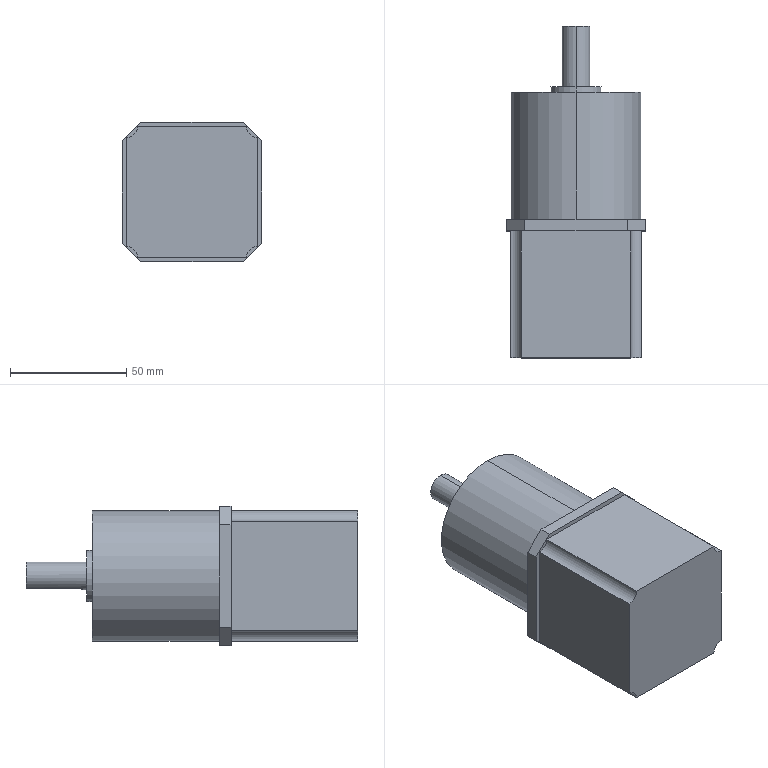Component | SolidWorks | LatestStepperMotor-1 | 1 solid | 49 faces | box 60 x 142.5 x 60 mm | volume 321837 mm3 | plane 21 | cylinder 20 | cone 8 | commonest cylinder face diameters 4.2 x8 9 x4 5 x2 12 x2 21.95 x2 56 x2 | material AISI 1045 Steel, Cold Drawn
build123d program:
from build123d import *

# Parameters (mm, degrees)
BOSS_EXTRUDE1_DEPTH   = 27.25
SKETCH2_W             = 60
SKETCH2_H             = 60
BOSS_EXTRUDE2_DEPTH   = 5
SKETCH3_R             = 28
BOSS_EXTRUDE3_DEPTH   = 54.5
SKETCH4_R             = 10.975
BOSS_EXTRUDE4_DEPTH   = 2.5
SKETCH5_R             = 6
BOSS_EXTRUDE5_DEPTH   = 26
CHAMFER1_SIZE         = 8
M5_TAPPED_HOLE1_D     = 4.2
M5_TAPPED_HOLE1_DEPTH = 13
M5_TAPPED_HOLE1_TIP   = 1.212
CUT_EXTRUDE1_DEPTH    = 3


with BuildPart() as part:
    # Sketch1 → Boss-Extrude1 (new, symmetric)
    with BuildSketch(Plane.XY):
        with BuildLine():
            Line((-23.5, 28), (23.5, 28))
            ThreePointArc((23.5, 28), (24.818, 24.818), (28, 23.5))
            Line((28, 23.5), (28, -23.5))
            ThreePointArc((28, -23.5), (24.818, -24.818), (23.5, -28))
            Line((23.5, -28), (-23.5, -28))
            ThreePointArc((-23.5, -28), (-24.818, -24.818), (-28, -23.5))
            Line((-28, -23.5), (-28, 23.5))
            ThreePointArc((-28, 23.5), (-24.818, 24.818), (-23.5, 28))
        make_face()
    extrude(amount=BOSS_EXTRUDE1_DEPTH, both=True)

    # Sketch2 → Boss-Extrude2 (add)
    with BuildSketch(Plane.XY.offset(27.25)):
        Rectangle(SKETCH2_W, SKETCH2_H)
    extrude(amount=BOSS_EXTRUDE2_DEPTH)

    # Sketch3 → Boss-Extrude3 (add)
    with BuildSketch(Plane.XY.offset(32.25)):
        Circle(SKETCH3_R)
    extrude(amount=BOSS_EXTRUDE3_DEPTH)

    # Sketch4 → Boss-Extrude4 (add)
    with BuildSketch(Plane.XY.offset(86.75)):
        Circle(SKETCH4_R)
    extrude(amount=BOSS_EXTRUDE4_DEPTH)

    # Sketch5 → Boss-Extrude5 (add)
    with BuildSketch(Plane.XY.offset(89.25)):
        with Locations(Location((0, 0, 0), (0, 0, 180))):
            Circle(SKETCH5_R)
    extrude(amount=BOSS_EXTRUDE5_DEPTH)

    # Chamfer1
    chamfer1_edges = [part.edges().sort_by_distance(p)[0] for p in [
        (30, -30, 29.75),
        (30, 30, 29.75),
        (-30, 30, 29.75),
        (-30, -30, 29.75),
    ]]
    chamfer(chamfer1_edges, length=CHAMFER1_SIZE)

    # M5 Tapped Hole1
    with Locations(Plane.XY.offset(86.75)):
        with Locations((-15.91, 15.91), (15.91, 15.91), (15.91, -15.91), (-15.91, -15.91)):
            Hole(M5_TAPPED_HOLE1_D / 2, depth=M5_TAPPED_HOLE1_DEPTH)
            with Locations((0, 0, -(M5_TAPPED_HOLE1_DEPTH + M5_TAPPED_HOLE1_TIP / 2))):  # 120° drill point
                Cone(0, M5_TAPPED_HOLE1_D / 2, M5_TAPPED_HOLE1_TIP, mode=Mode.SUBTRACT)

    # Sketch9 → Cut-Extrude1 (cut)
    with BuildSketch(Plane(origin=(6, 0, 0), x_dir=(0, 0, -1), z_dir=(1, 0, 0))):
        with BuildLine():
            Line((-115.25, 2.5), (-92.75, 2.5))
            ThreePointArc((-92.75, 2.5), (-90.25, 0), (-92.75, -2.5))
            Line((-92.75, -2.5), (-115.25, -2.5))
            ThreePointArc((-115.25, -2.5), (-117.75, 0), (-115.25, 2.5))
        make_face()
    extrude(amount=-CUT_EXTRUDE1_DEPTH, mode=Mode.SUBTRACT)


solid = part.part

# Placed as in the assembly
solid = solid.moved(Location((-96.534, 21.516, -166.507), (-90, 0, 90)))